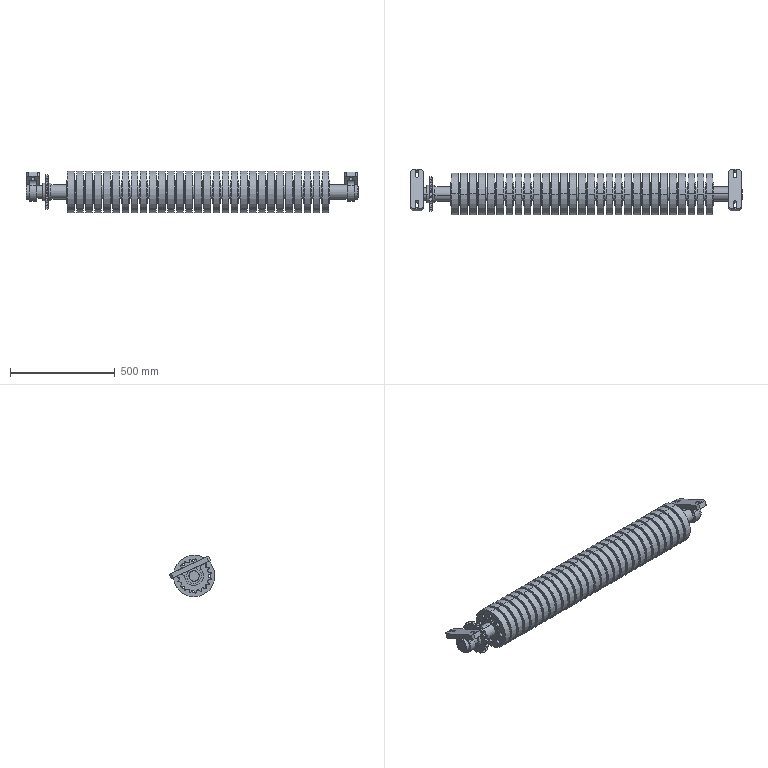Assembly | SolidWorks | mm | 93 component files | 93 solids | 1734 faces | box 1587 x 217.7 x 198.68 mm | volume 28490596 mm3 | cylinder 1069 | plane 371 | cone 234 | torus 60 | commonest cylinder face diameters 20 x240 30 x224 60 x164 95 x118 68 x60 109 x60 198.68 x58 15.88 x44
Bill of materials:
19ToothSprocket | 1 |  | Spur-type toothed sprocket disc with a central bore, a single keyway, and a cylindrical hub that protrudes on both faces of the toothed plate.
6012 | 29 |  | Thick plain annular ring (washer or spacer form) with flat parallel faces and a concentric through bore.
DrivePulleyShaft | 1 |  | Long slender cylindrical shaft with a reduced-diameter stepped journal at each end.
SpindleSleeve1 | 1 |  | Thin-walled cylindrical tube or sleeve, open at both ends, with length longer than its outer diameter.
SpindleSleeve2 | 28 |  | Narrow thin-walled annular ring (short band) with a rectangular cross-section.
SpindleSleeve3 | 1 |  | Thin-walled cylindrical tube or sleeve, open at both ends, with length a little longer than its diameter.
SpindleSleeve4 | 1 |  | Short cylindrical ring or bushing with a moderate wall thickness and length shorter than its diameter.
SynchronousDrivenPulley | 15 |  | Annular flange with a central bore, eight evenly spaced through holes on a bolt circle, and a short raised concentric spigot or boss around the bore.
SynchronousDrivePulley | 14 |  | Flat circular disc with a central keyed bore and eight evenly spaced round through holes around it.
Z90510 | 2 |  | Bracket made of a rectangular mounting plate with chamfered corners and two elongated slots, joined by a web to an offset cylindrical boss with a through bore (pillow-block-like form).
Mates:
1. concentric | DrivePulleyShaft-1 face at (661.803, 34.532, 0) dir (-1, 0, 0) r 30 | SynchronousDrivePulley-1 face at (534.553, 34.532, 0) dir (-1, 0, 0) r 30
2. coincident | DrivePulleyShaft-1 face at (-627.697, 57.532, -9) dir (0, 0, 1) | SynchronousDrivePulley-1 face at (534.553, 69.932, -9) dir (0, 0, 1)
3. concentric | DrivePulleyShaft-1 face at (-789.197, 34.532, 0) dir (-1, 0, 0) r 25 | Z90510-2 face at (-869.297, 34.532, 0) dir (1, 0, 0) r 25
4. concentric | DrivePulleyShaft-1 face at (716.803, 34.532, 0) dir (-1, 0, 0) r 25 | Z90510-1 face at (715.903, 34.532, 0) dir (-1, 0, 0) r 25
5. concentric | SynchronousDrivenPulley-1 face at (582.053, 34.532, 0) dir (-1, 0, 0) r 47.5 | 6012-1 face at (581.303, 34.532, 0) dir (-1, 0, 0) r 30
6. concentric | 6012-1 face at (581.303, 34.532, 0) dir (-1, 0, 0) r 30 | 6012-2 face at (560.803, 34.532, 0) dir (-1, 0, 0) r 30
7. concentric | DrivePulleyShaft-1 face at (661.803, 34.532, 0) dir (-1, 0, 0) r 30 | SynchronousDrivenPulley-1 face at (578.053, 34.532, 0) dir (-1, 0, 0) r 99.34
8. concentric | DrivePulleyShaft-1 face at (661.803, 34.532, 0) dir (-1, 0, 0) r 30 | SpindleSleeve1-1 face at (664.303, 34.532, 0) dir (-1, 0, 0) r 34
9. coincident | SpindleSleeve1-1 face at (581.303, 34.532, 0) dir (-1, 0, 0) | 6012-1 face at (581.303, 34.532, 0) dir (1, 0, 0)
10. distance | SynchronousDrivePulley-1 face at (534.553, 34.532, 0) dir (1, 0, 0) | SynchronousDrivenPulley-1 face at (546.053, 34.532, 0) dir (-1, 0, 0)
11. concentric | DrivePulleyShaft-1 face at (661.803, 34.532, 0) dir (-1, 0, 0) r 30 | SpindleSleeve2-1 face at (534.553, 34.532, 0) dir (1, 0, 0) r 30
12. coincident | SynchronousDrivePulley-1 face at (534.553, 34.532, 0) dir (1, 0, 0) | SpindleSleeve2-1 face at (534.553, 34.532, 0) dir (-1, 0, 0)
13. concentric | DrivePulleyShaft-1 face at (661.803, 34.532, 0) dir (-1, 0, 0) r 30 | SpindleSleeve2-31 face at (494.303, 34.532, 0) dir (1, 0, 0) r 34
14. coincident | SynchronousDrivePulley-1 face at (502.553, 34.532, 0) dir (-1, 0, 0) | SpindleSleeve2-31 face at (502.553, 34.532, 0) dir (1, 0, 0)
15. concentric | DrivePulleyShaft-1 face at (-749.197, 34.532, 0) dir (-1, 0, 0) r 26 | 19ToothSprocket-1 face at (-791.197, 34.532, 0) dir (1, 0, 0) r 26
16. coincident | DrivePulleyShaft-1 face at (-789.197, 54.532, -8) dir (0, 0, 1) | 19ToothSprocket-1 face at (-791.197, 64.832, -8) dir (0, 0, 1)
17. concentric | DrivePulleyShaft-1 face at (-789.197, 34.532, 0) dir (-1, 0, 0) r 25 | SpindleSleeve4-1 face at (-791.197, 34.532, 0) dir (-1, 0, 0) r 30
18. coincident | 19ToothSprocket-1 face at (-791.197, 34.532, 0) dir (-1, 0, 0) | SpindleSleeve4-1 face at (-791.197, 34.532, 0) dir (1, 0, 0)
19. concentric | DrivePulleyShaft-1 face at (-789.197, 34.532, 0) dir (-1, 0, 0) r 25 | Z90510-2 face at (-869.297, 34.532, 0) dir (1, 0, 0) r 25
20. coincident | SpindleSleeve4-1 face at (-817.697, 34.532, 0) dir (-1, 0, 0) | Z90510-2 face at (-817.697, 34.532, 0) dir (1, 0, 0)
21. coincident | Z90510-1 face at (713.803, 152.89, 8.892) dir (0, 0.4149, 0.9099) | Z90510-2 face at (-867.197, -36.36, 95.196) dir (0, 0.4149, 0.9099)
22. concentric | DrivePulleyShaft-1 face at (661.803, 34.532, 0) dir (-1, 0, 0) r 30 | SynchronousDrivenPulley-16 face at (-635.947, 34.532, 0) dir (-1, 0, 0) r 47.5
23. concentric | DrivePulleyShaft-1 face at (661.803, 34.532, 0) dir (-1, 0, 0) r 30 | SpindleSleeve3-1 face at (-751.197, 34.532, 0) dir (1, 0, 0) r 34
24. coincident | 19ToothSprocket-1 face at (-751.197, 34.532, 0) dir (1, 0, 0) | SpindleSleeve3-1 face at (-751.197, 34.532, 0) dir (-1, 0, 0)
25. distance | SynchronousDrivePulley-14 face at (-628.447, 34.532, 0) dir (-1, 0, 0) | SynchronousDrivenPulley-16 face at (-639.947, 34.532, 0) dir (1, 0, 0)
26. distance | 6012-1 face at (581.303, 34.532, 0) dir (1, 0, 0) | SynchronousDrivenPulley-1 face at (582.053, 34.532, 0) dir (1, 0, 0)
27. distance | SynchronousDrivenPulley-1 face at (542.053, 34.532, 0) dir (-1, 0, 0) | 6012-2 face at (542.803, 34.532, 0) dir (-1, 0, 0)
28. distance | SynchronousDrivenPulley-16 face at (-675.947, 34.532, 0) dir (-1, 0, 0) | 6012-31 face at (-675.197, 34.532, 0) dir (-1, 0, 0)
29. concentric | SynchronousDrivenPulley-16 face at (-635.947, 34.532, 0) dir (-1, 0, 0) r 47.5 | 6012-31 face at (-657.197, 34.532, 0) dir (-1, 0, 0) r 47.5
30. distance | Z90510-1 face at (715.903, 34.532, 0) dir (1, 0, 0) | DrivePulleyShaft-1 face at (716.803, 34.532, 0) dir (1, 0, 0)
31. coincident | SpindleSleeve1-1 face at (664.303, 34.532, 0) dir (1, 0, 0) | Z90510-1 face at (664.303, 34.532, 0) dir (-1, 0, 0)
32. coincident | SpindleSleeve3-1 face at (-675.197, 34.532, 0) dir (1, 0, 0) | 6012-31 face at (-675.197, 34.532, 0) dir (-1, 0, 0)